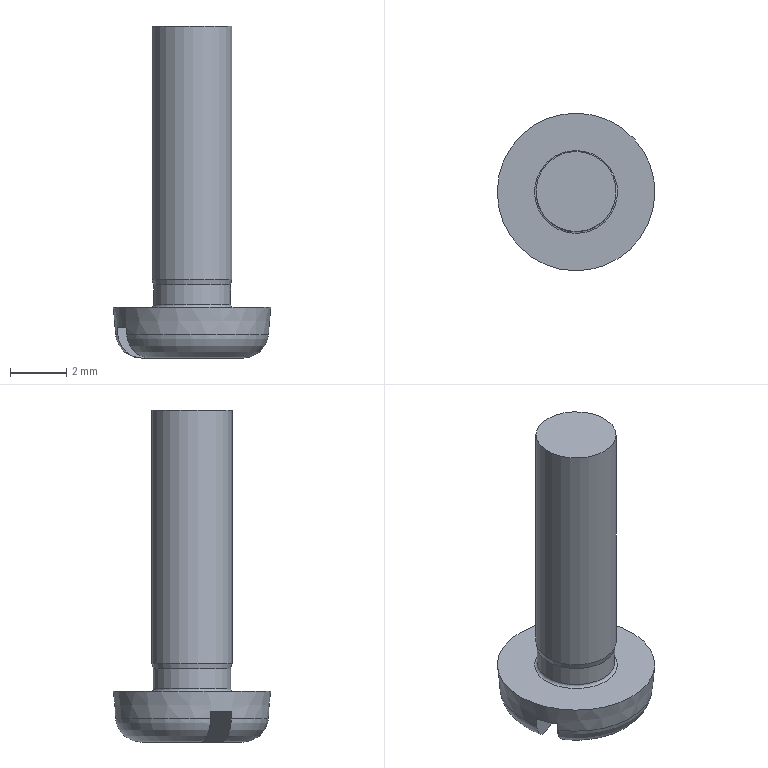Component | NX | 08_SCREW | 1 solid | 14 faces | volume 98 mm3 | plane 7 | torus 3 | cone 2 | cylinder 2 | commonest cylinder face diameters 2.747 x1 2.847 x1